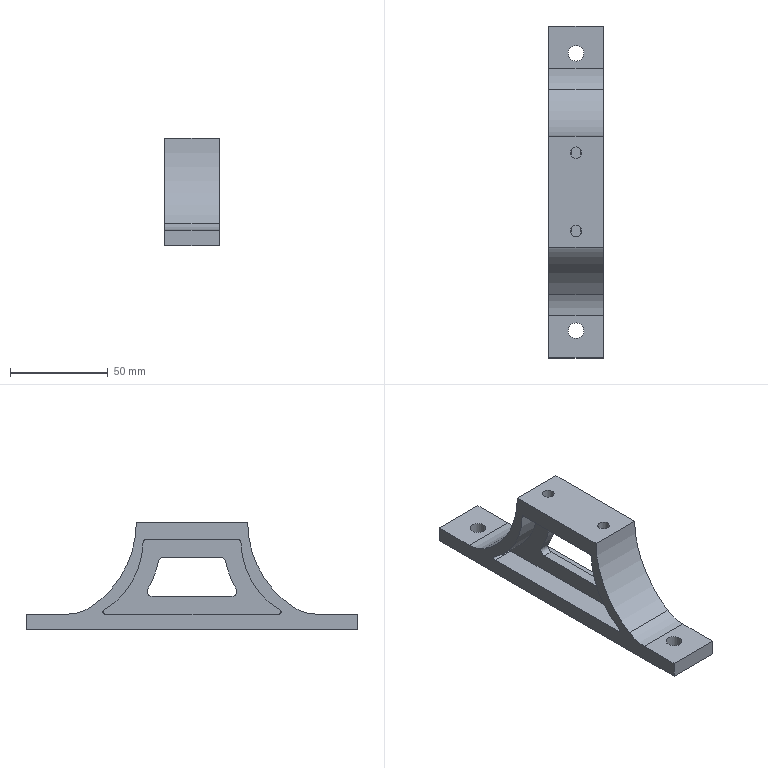Component | NX | SUPPORT_PLATFORM | 1 solid | 44 faces | volume 74883 mm3 | cylinder 26 | plane 18 | commonest cylinder face diameters 2 x8 85 x4 5 x4 103.956 x2 40 x2 103 x2 8 x2 6 x2